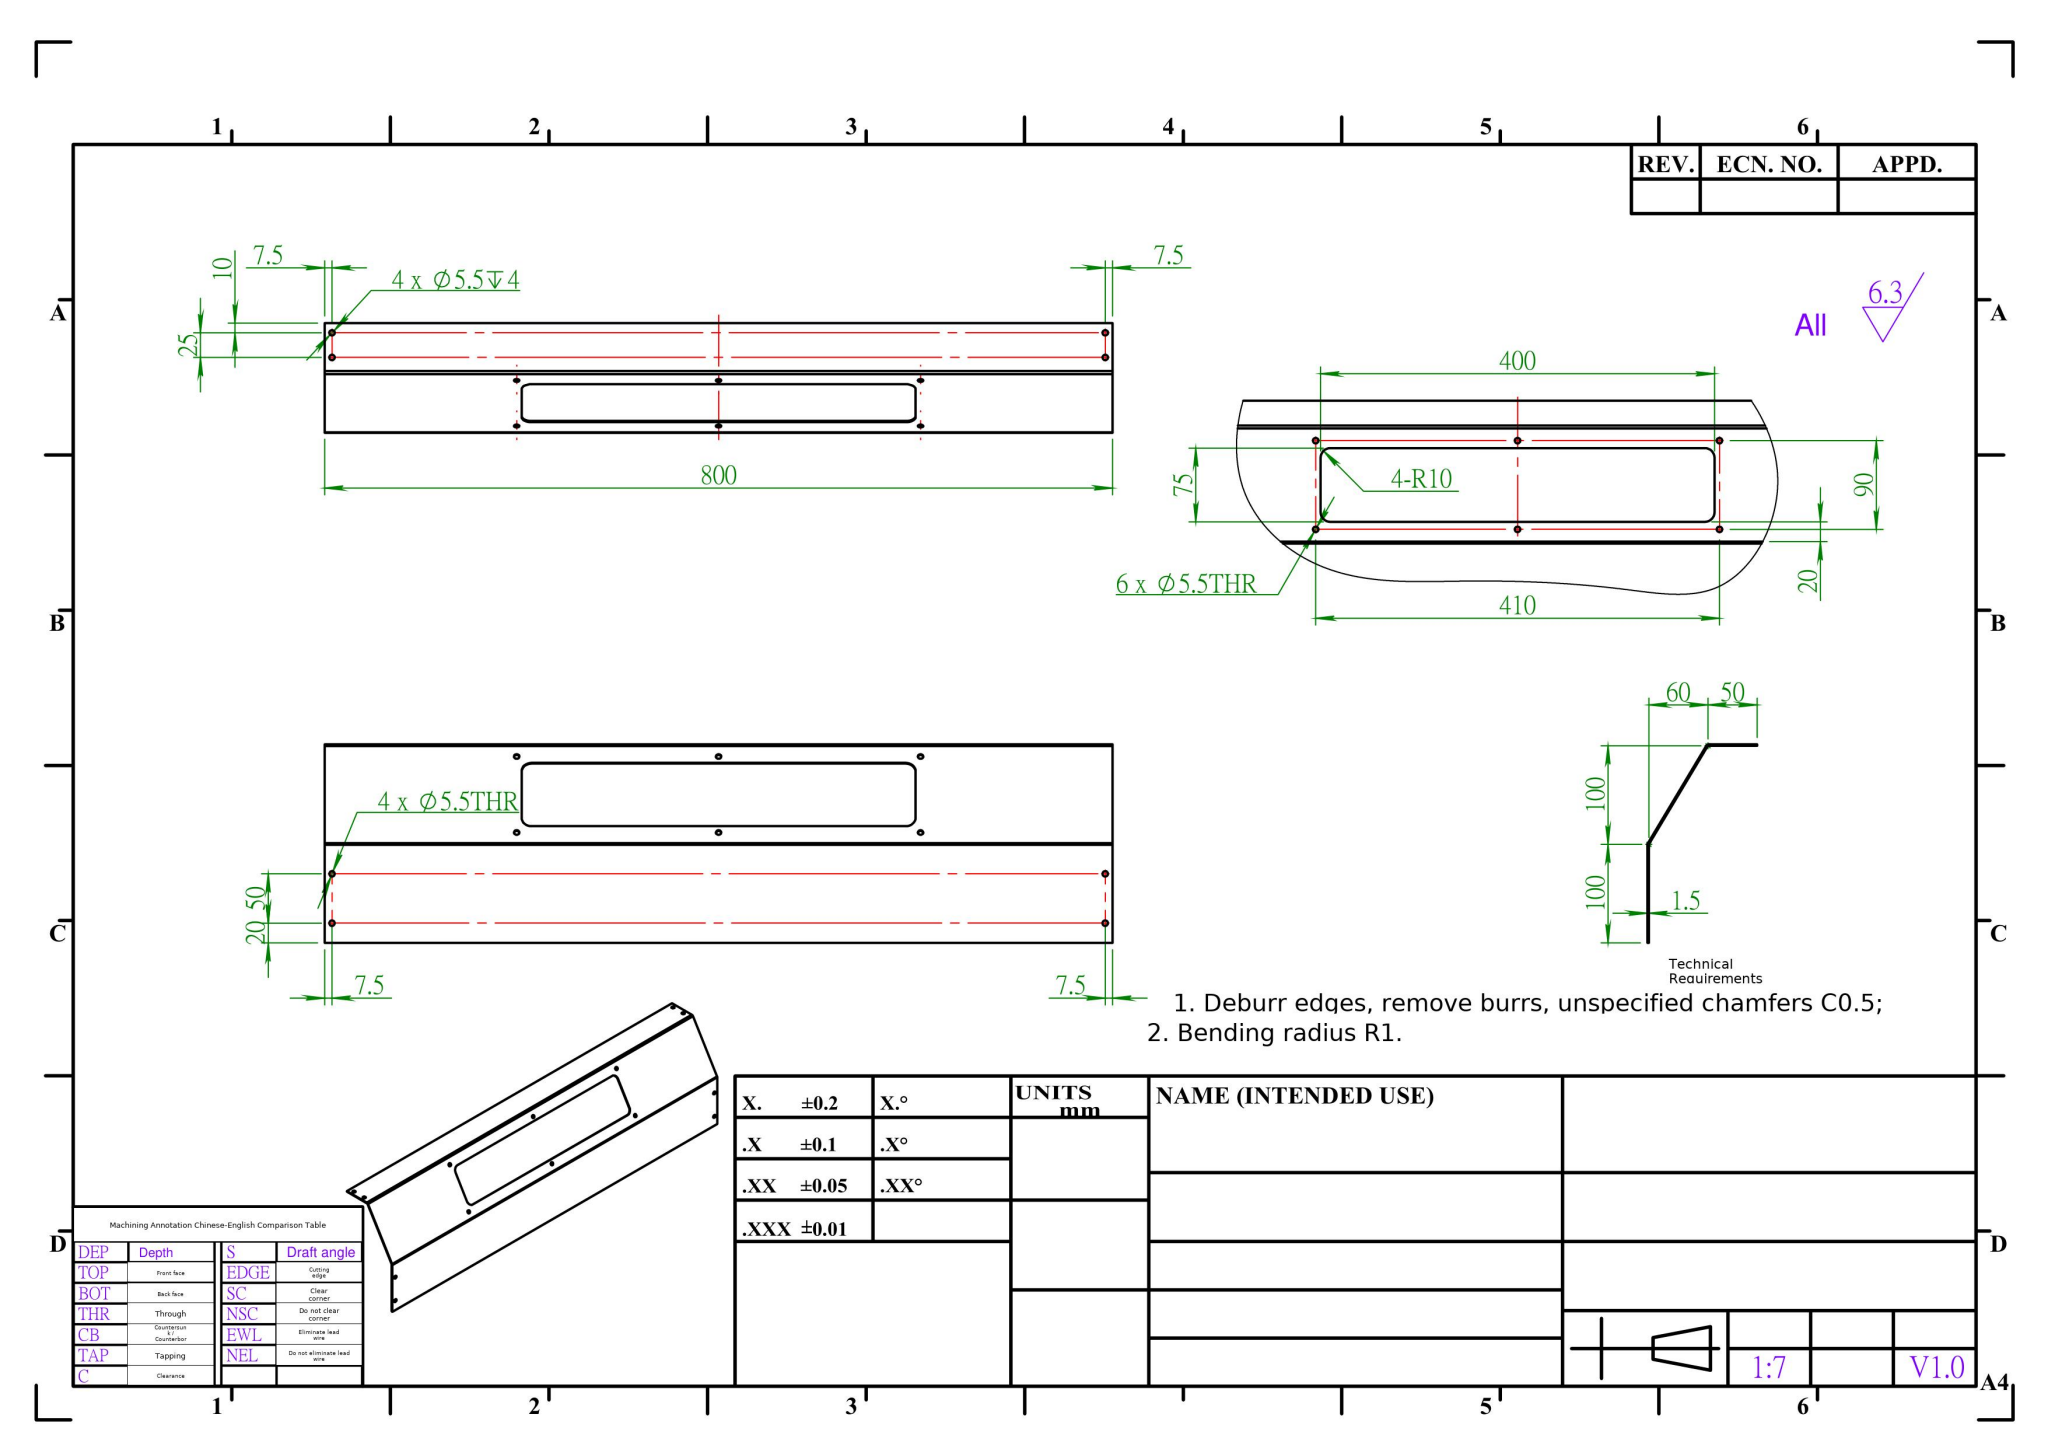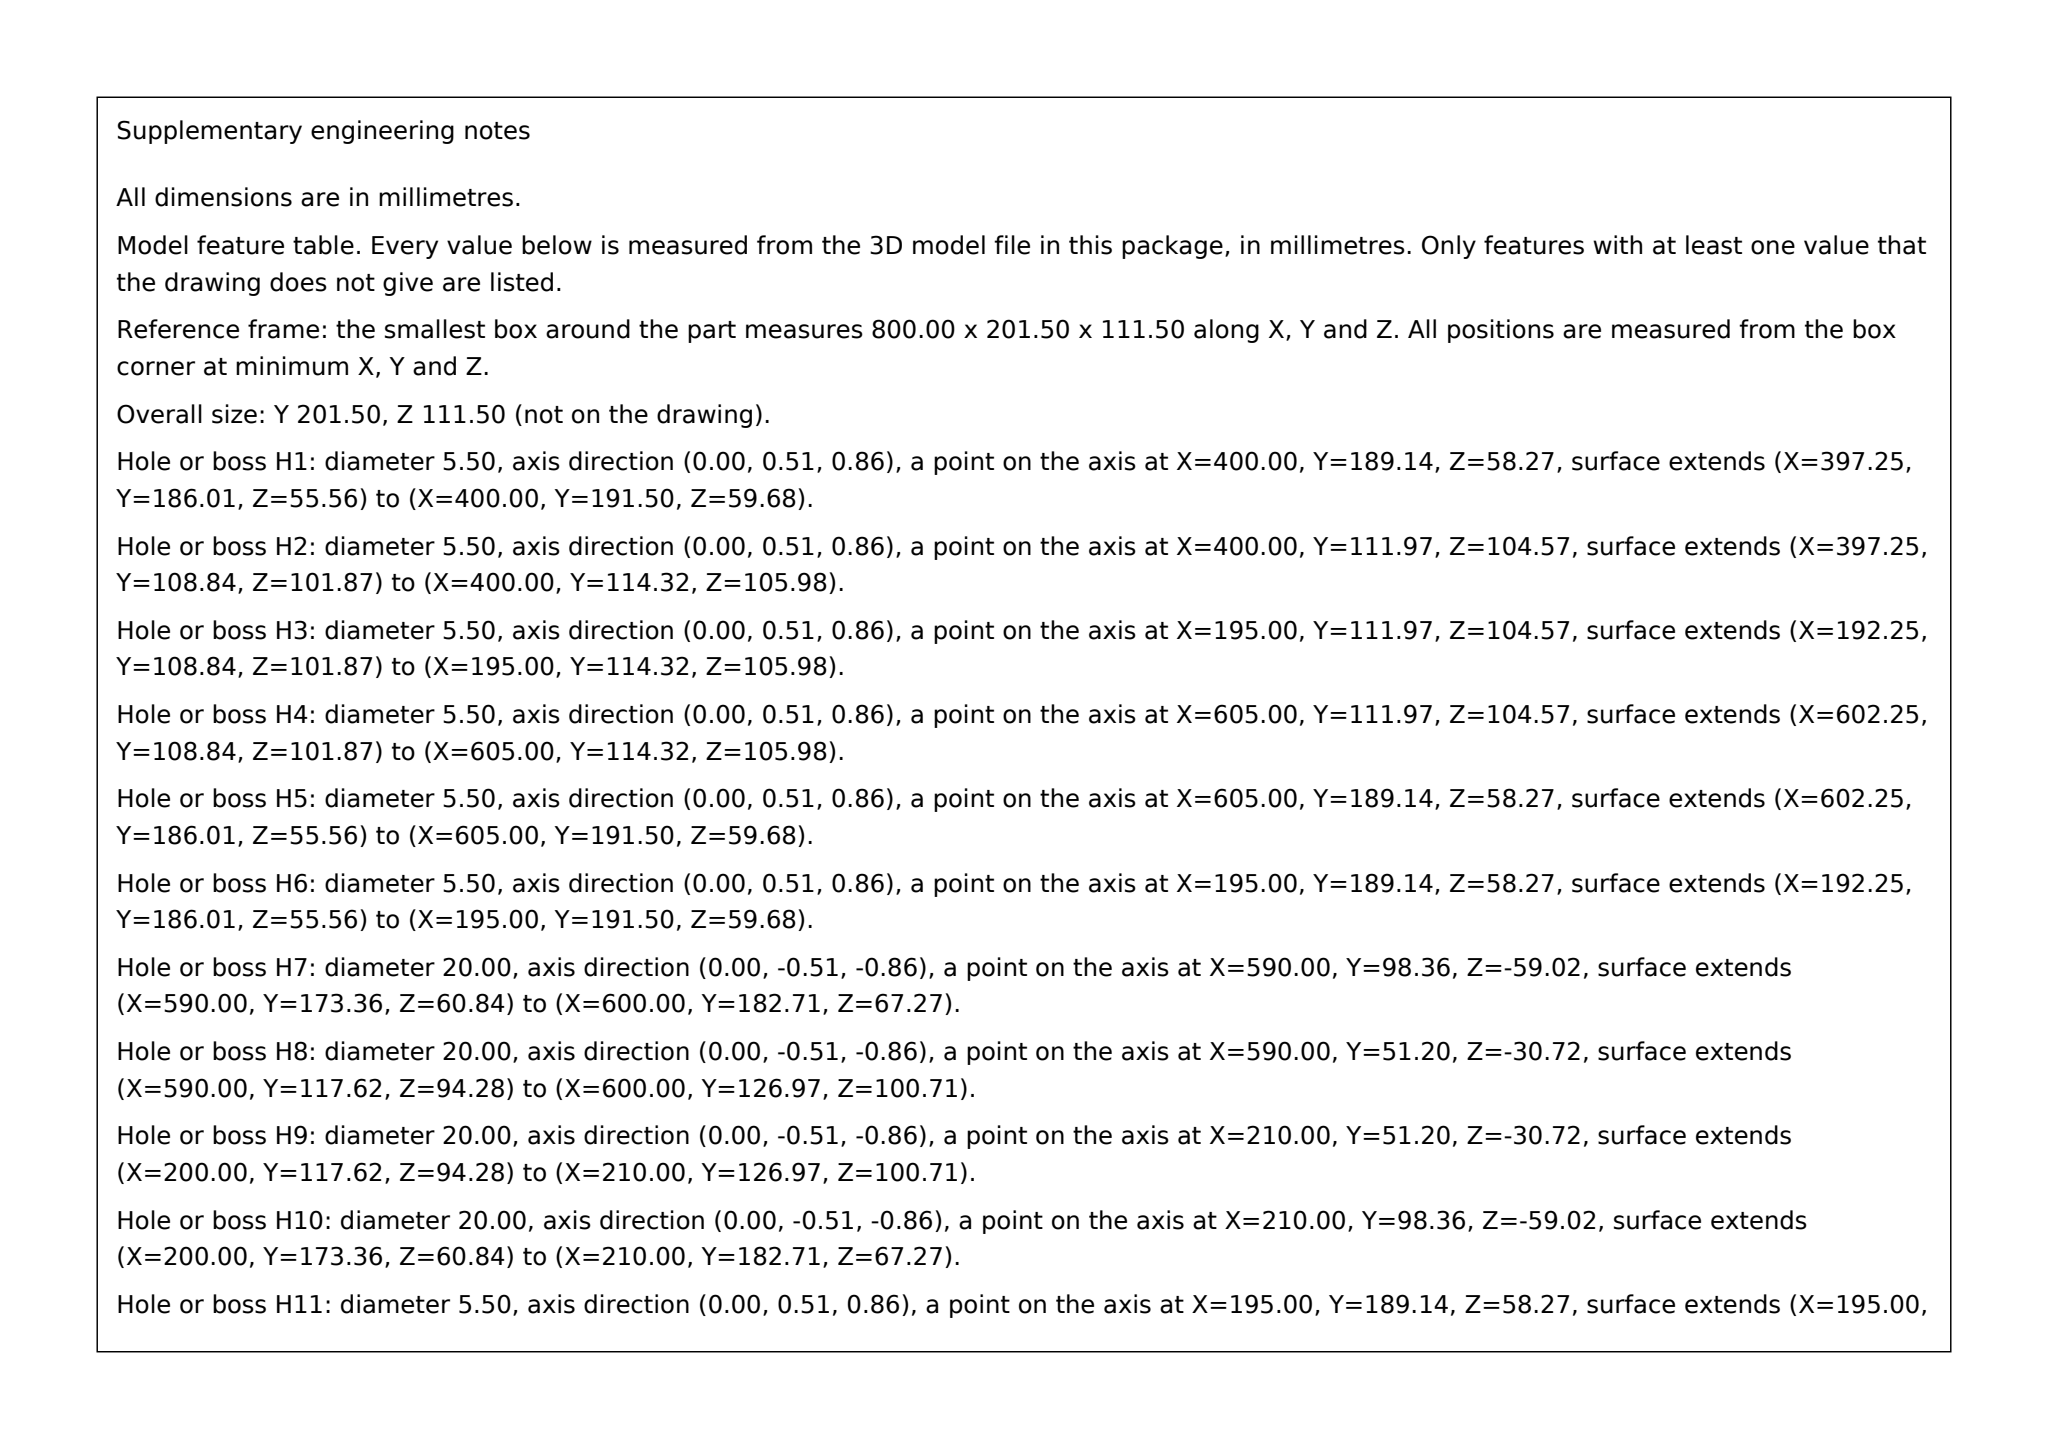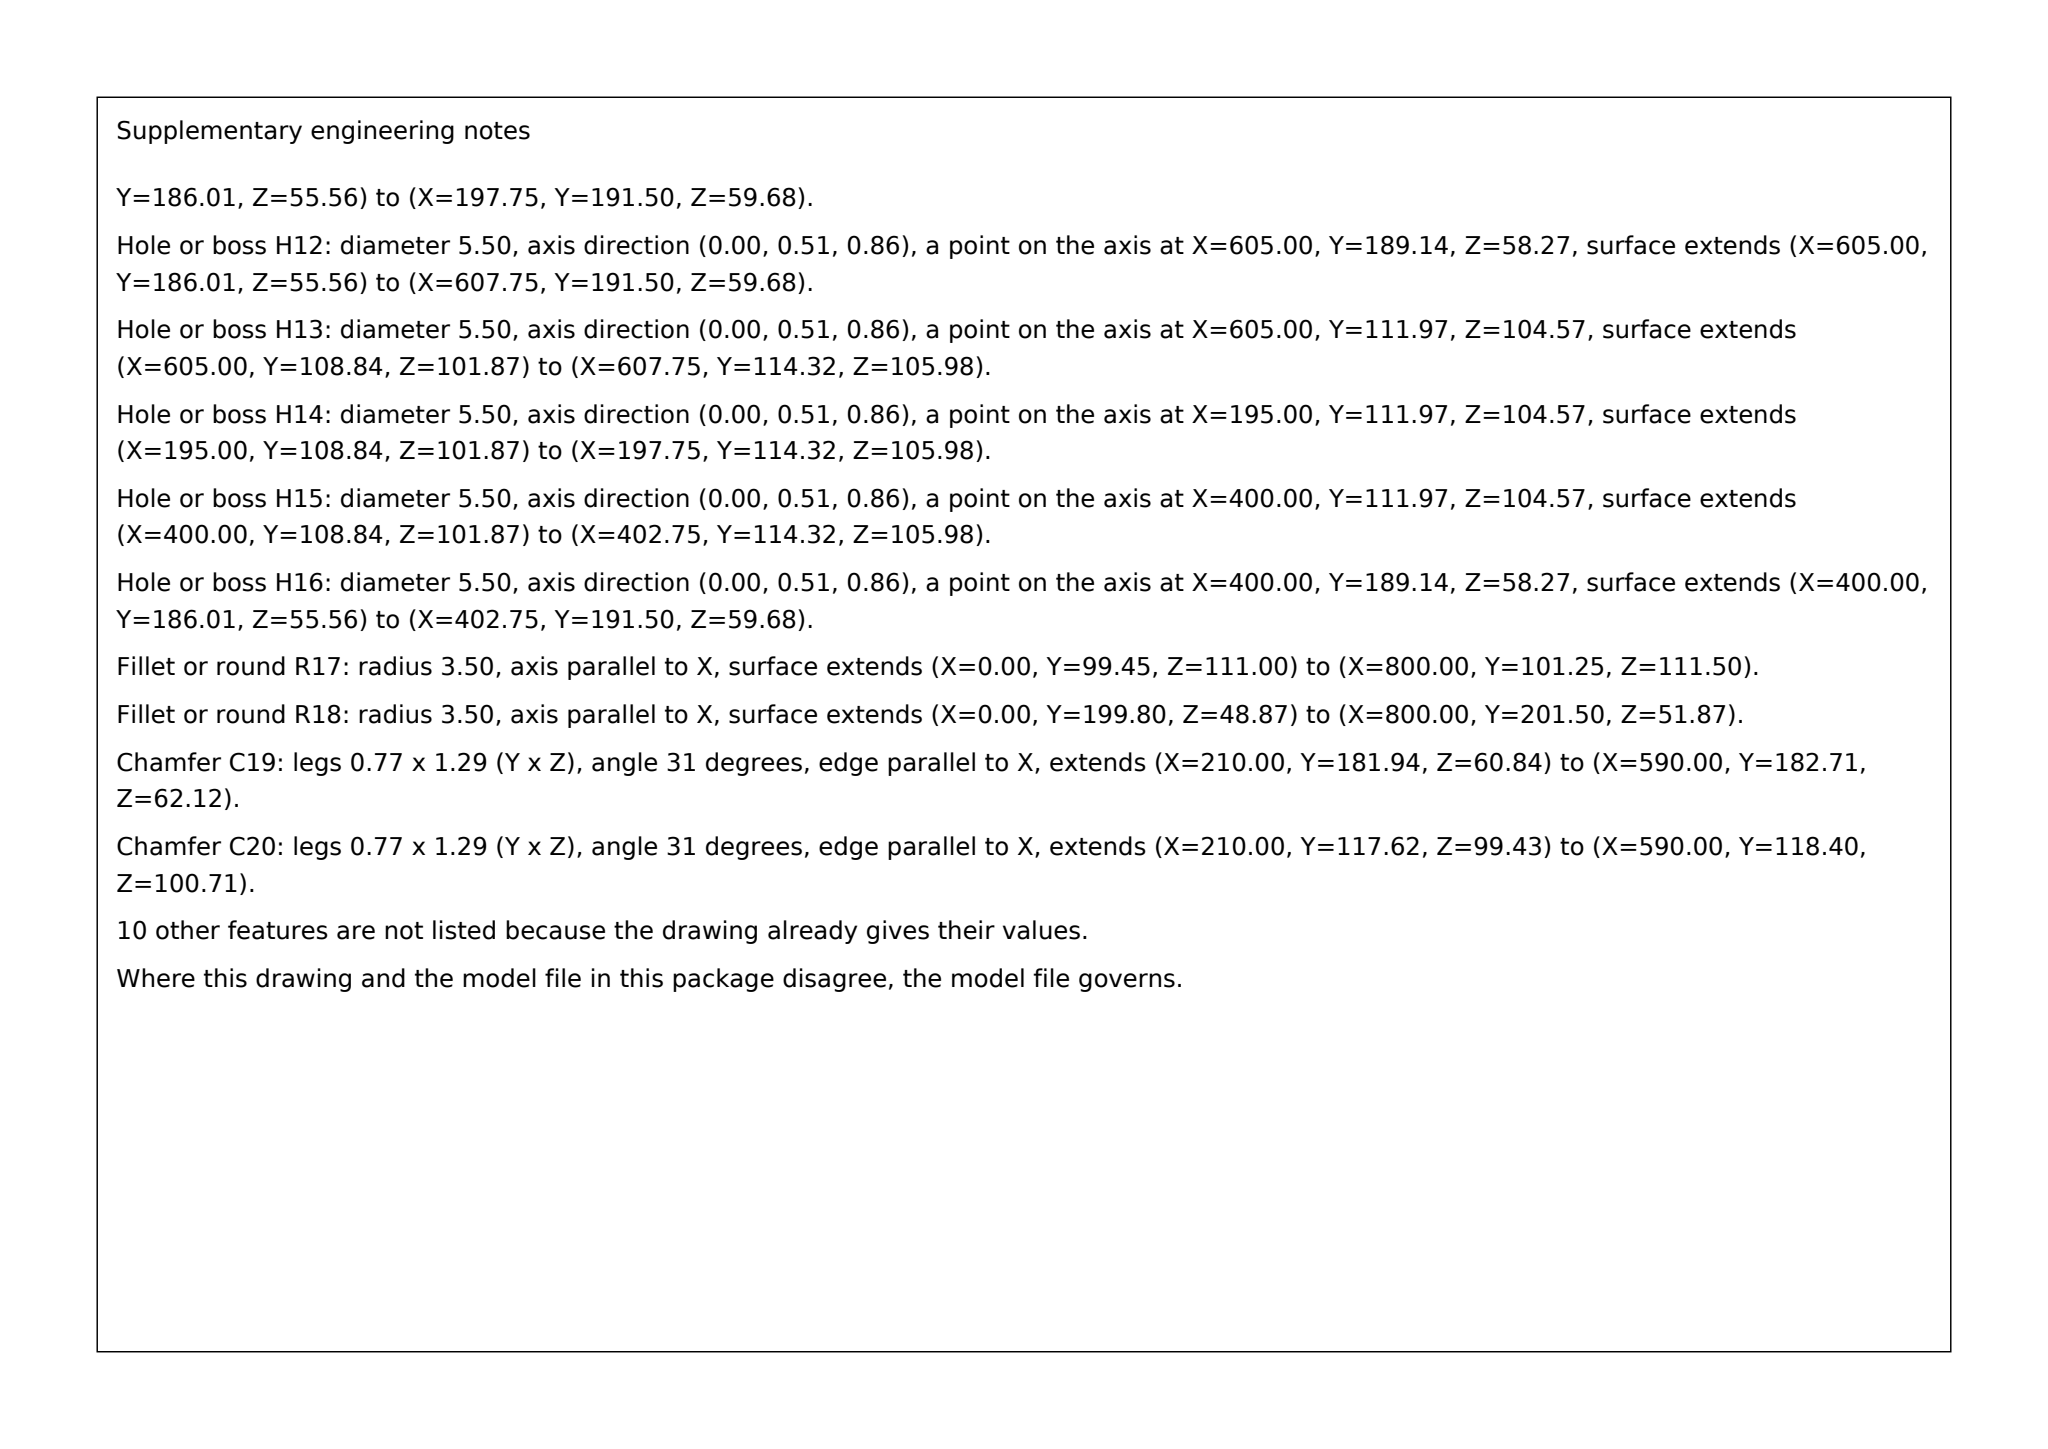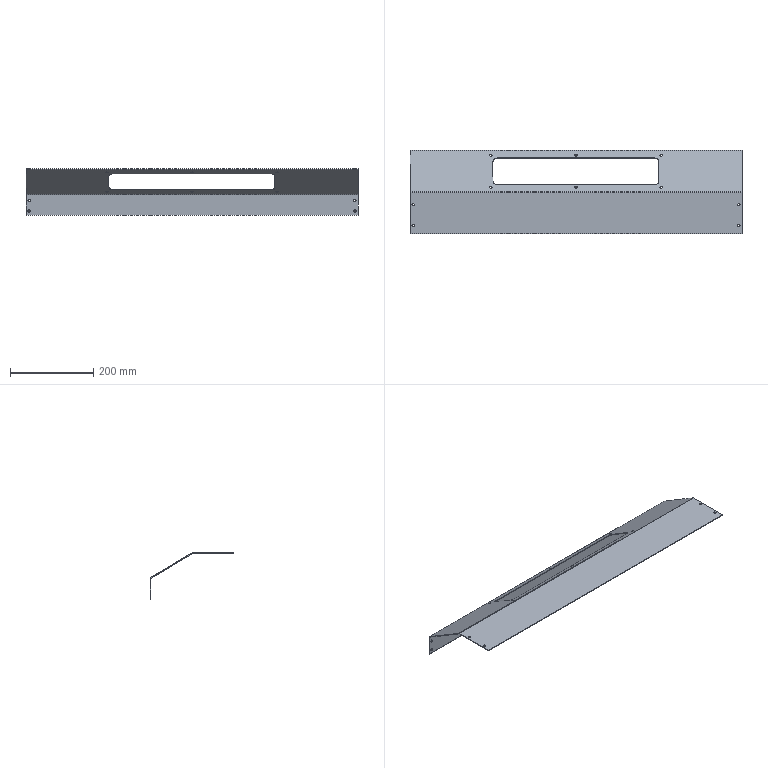Part | SolidWorks | mm | 1 solid | 58 faces | box 800 x 201.5 x 111.5 mm | volume 275709 mm3 | cylinder 36 | plane 22 | commonest cylinder face diameters 5.5 x28 20 x4 7 x2 4 x2